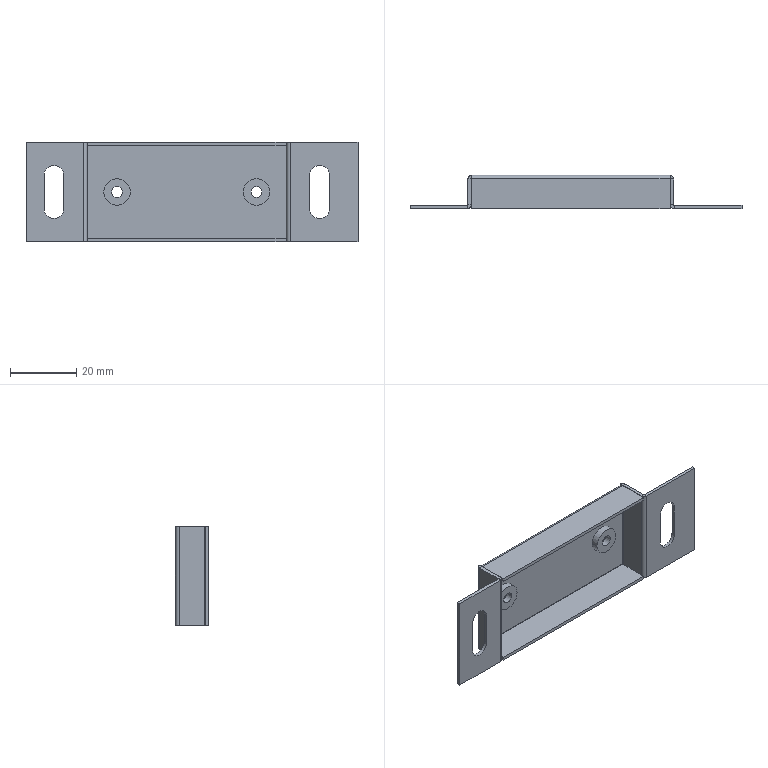Component | SolidWorks | BearingHousingBracket-1 | 1 solid | 82 faces | volume 4499 mm3 | plane 54 | cylinder 28 | commonest cylinder face diameters 2.2 x6 0.2 x6 3.3 x4 8 x4 5.4 x4 6 x4